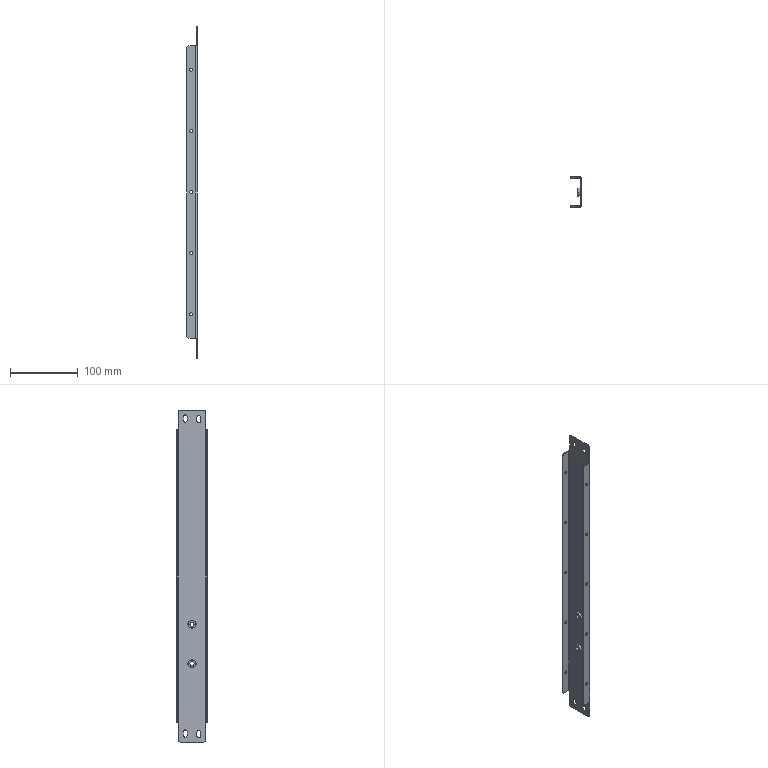Component | SolidWorks | MoldedCaseMountingBeamOne100-21 | 1 solid | 88 faces | volume 48825 mm3 | cylinder 52 | plane 32 | cone 4 | commonest cylinder face diameters 4.5 x20 6 x12 5.5 x12 12 x4 4.473 x2 1.473 x2